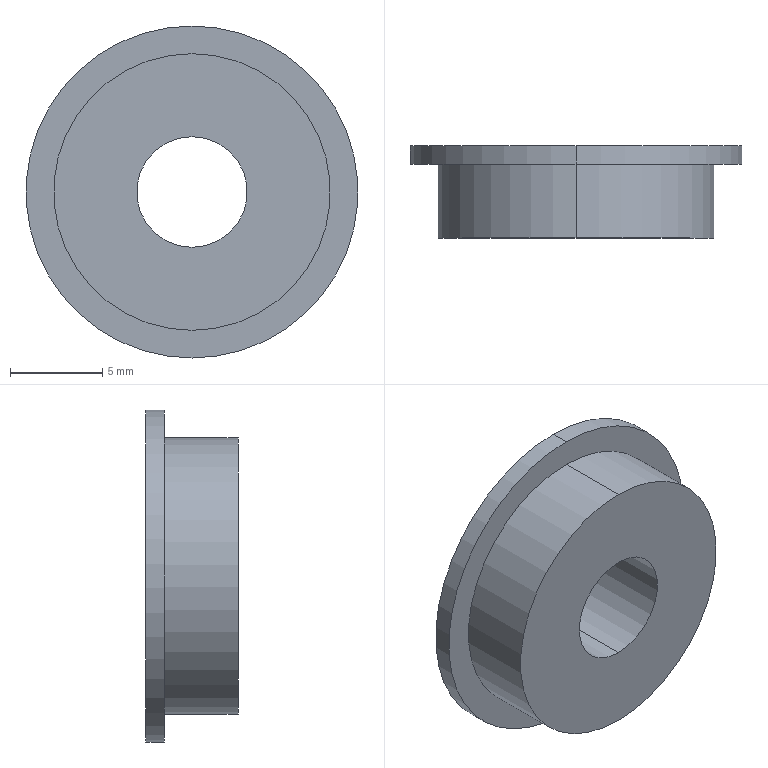Component | SolidWorks | 6 15 5 F-2 | 1 solid | 9 faces | box 18 x 5 x 18 mm | volume 820 mm3 | cylinder 6 | plane 3 | commonest cylinder face diameters 18 x2 6 x2 15 x2
build123d program:
from build123d import *

# Parameters (mm, degrees)
SKETCH1_R           = 7.5
SKETCH1_R_2         = 3
BOSS_EXTRUDE1_DEPTH = 5
BOSS_EXTRUDE2_START = -1
SKETCH2_R           = 9
SKETCH2_R_2         = 3
BOSS_EXTRUDE2_DEPTH = 1


with BuildPart() as part:
    # Sketch1 → Boss-Extrude1 (new body)
    with BuildSketch(Plane(origin=(0, 0, 0), x_dir=(1, 0, 0), z_dir=(0, 1, 0))):
        with Locations(Location((0, 0, 0), (0, 0, 270))):
            Circle(SKETCH1_R)
        with Locations(Location((0, 0, 0), (0, 0, 270))):
            Circle(SKETCH1_R_2, mode=Mode.SUBTRACT)
    extrude(amount=BOSS_EXTRUDE1_DEPTH)

    # Sketch2 → Boss-Extrude2 (add)
    with BuildSketch(Plane(origin=(0, 5, 0), x_dir=(1, 0, 0), z_dir=(0, 1, 0)).offset(BOSS_EXTRUDE2_START)):
        with Locations(Location((0, 0, 0), (0, 0, 270))):
            Circle(SKETCH2_R)
        with Locations(Location((0, 0, 0), (0, 0, 270))):
            Circle(SKETCH2_R_2, mode=Mode.SUBTRACT)
    extrude(amount=BOSS_EXTRUDE2_DEPTH)


solid = part.part

# Placed as in the assembly
solid = solid.moved(Location((0.3183, -14.6, 37), (0, 0, 0)))
STEP:
#1=COLOUR_RGB('',0.7922,0.8196,0.9333);
#2=FILL_AREA_STYLE_COLOUR('',#1);
#3=FILL_AREA_STYLE('',(#2));
#4=SURFACE_STYLE_FILL_AREA(#3);
#5=SURFACE_SIDE_STYLE('',(#4));
#6=SURFACE_STYLE_USAGE(.BOTH.,#5);
#7=PRESENTATION_STYLE_ASSIGNMENT((#6));
#8=CARTESIAN_POINT('',(0.01253,-0.4173,1.811));
#9=VERTEX_POINT('',#8);
#10=CARTESIAN_POINT('',(0.01253,-0.4173,1.102));
#11=VERTEX_POINT('',#10);
#12=CARTESIAN_POINT('',(0.01253,-0.4173,1.457));
#13=DIRECTION('',(0.,1.,0.));
#14=DIRECTION('',(0.,0.,1.));
#15=AXIS2_PLACEMENT_3D('',#12,#13,#14);
#16=CIRCLE('',#15,0.3543);
#17=EDGE_CURVE('',#9,#11,#16,.T.);
#18=ORIENTED_EDGE('',*,*,#17,.T.);
#19=CARTESIAN_POINT('',(0.01253,-0.378,1.102));
#20=VERTEX_POINT('',#19);
#21=CARTESIAN_POINT('',(0.01253,-0.4173,1.102));
#22=DIRECTION('',(0.,1.,0.));
#23=VECTOR('',#22,39.37);
#24=LINE('',#21,#23);
#25=EDGE_CURVE('',#11,#20,#24,.T.);
#26=ORIENTED_EDGE('',*,*,#25,.T.);
#27=CARTESIAN_POINT('',(0.01253,-0.378,1.811));
#28=VERTEX_POINT('',#27);
#29=CARTESIAN_POINT('',(0.01253,-0.378,1.457));
#30=DIRECTION('',(0.,1.,0.));
#31=DIRECTION('',(0.,0.,1.));
#32=AXIS2_PLACEMENT_3D('',#29,#30,#31);
#33=CIRCLE('',#32,0.3543);
#34=EDGE_CURVE('',#28,#20,#33,.T.);
#35=ORIENTED_EDGE('',*,*,#34,.F.);
#36=CARTESIAN_POINT('',(0.01253,-0.4173,1.811));
#37=DIRECTION('',(0.,1.,0.));
#38=VECTOR('',#37,39.37);
#39=LINE('',#36,#38);
#40=EDGE_CURVE('',#9,#28,#39,.T.);
#41=ORIENTED_EDGE('',*,*,#40,.F.);
#42=EDGE_LOOP('',(#18,#26,#35,#41));
#43=FACE_OUTER_BOUND('',#42,.T.);
#44=CARTESIAN_POINT('',(0.01253,-0.4173,1.457));
#45=DIRECTION('',(0.,1.,0.));
#46=DIRECTION('',(0.,0.,1.));
#47=AXIS2_PLACEMENT_3D('',#44,#45,#46);
#48=CYLINDRICAL_SURFACE('',#47,0.3543);
#49=ADVANCED_FACE('',(#43),#48,.T.);
#50=CARTESIAN_POINT('',(0.01253,-0.378,1.339));
#51=VERTEX_POINT('',#50);
#52=CARTESIAN_POINT('',(0.01253,-0.378,1.575));
#53=VERTEX_POINT('',#52);
#54=CARTESIAN_POINT('',(0.01253,-0.378,1.457));
#55=DIRECTION('',(0.,1.,0.));
#56=DIRECTION('',(0.,0.,1.));
#57=AXIS2_PLACEMENT_3D('',#54,#55,#56);
#58=CIRCLE('',#57,0.1181);
#59=EDGE_CURVE('',#51,#53,#58,.T.);
#60=ORIENTED_EDGE('',*,*,#59,.T.);
#61=CARTESIAN_POINT('',(0.01253,-0.5748,1.575));
#62=VERTEX_POINT('',#61);
#63=CARTESIAN_POINT('',(0.01253,-0.378,1.575));
#64=DIRECTION('',(0.,-1.,0.));
#65=VECTOR('',#64,39.37);
#66=LINE('',#63,#65);
#67=EDGE_CURVE('',#53,#62,#66,.T.);
#68=ORIENTED_EDGE('',*,*,#67,.T.);
#69=CARTESIAN_POINT('',(0.01253,-0.5748,1.339));
#70=VERTEX_POINT('',#69);
#71=CARTESIAN_POINT('',(0.01253,-0.5748,1.457));
#72=DIRECTION('',(0.,1.,0.));
#73=DIRECTION('',(0.,0.,1.));
#74=AXIS2_PLACEMENT_3D('',#71,#72,#73);
#75=CIRCLE('',#74,0.1181);
#76=EDGE_CURVE('',#70,#62,#75,.T.);
#77=ORIENTED_EDGE('',*,*,#76,.F.);
#78=CARTESIAN_POINT('',(0.01253,-0.378,1.339));
#79=DIRECTION('',(0.,-1.,0.));
#80=VECTOR('',#79,39.37);
#81=LINE('',#78,#80);
#82=EDGE_CURVE('',#51,#70,#81,.T.);
#83=ORIENTED_EDGE('',*,*,#82,.F.);
#84=EDGE_LOOP('',(#60,#68,#77,#83));
#85=FACE_OUTER_BOUND('',#84,.T.);
#86=CARTESIAN_POINT('',(0.01253,-0.378,1.457));
#87=DIRECTION('',(0.,-1.,0.));
#88=DIRECTION('',(0.,0.,-1.));
#89=AXIS2_PLACEMENT_3D('',#86,#87,#88);
#90=CYLINDRICAL_SURFACE('',#89,0.1181);
#91=ADVANCED_FACE('',(#85),#90,.F.);
#92=CARTESIAN_POINT('',(0.01253,-0.4173,1.752));
#93=VERTEX_POINT('',#92);
#94=CARTESIAN_POINT('',(0.01253,-0.4173,1.161));
#95=VERTEX_POINT('',#94);
#96=CARTESIAN_POINT('',(0.01253,-0.4173,1.457));
#97=DIRECTION('',(0.,1.,0.));
#98=DIRECTION('',(0.,0.,1.));
#99=AXIS2_PLACEMENT_3D('',#96,#97,#98);
#100=CIRCLE('',#99,0.2953);
#101=EDGE_CURVE('',#93,#95,#100,.T.);
#102=ORIENTED_EDGE('',*,*,#101,.F.);
#103=CARTESIAN_POINT('',(0.01253,-0.5748,1.752));
#104=VERTEX_POINT('',#103);
#105=CARTESIAN_POINT('',(0.01253,-0.378,1.752));
#106=DIRECTION('',(0.,-1.,0.));
#107=VECTOR('',#106,39.37);
#108=LINE('',#105,#107);
#109=EDGE_CURVE('',#93,#104,#108,.T.);
#110=ORIENTED_EDGE('',*,*,#109,.T.);
#111=CARTESIAN_POINT('',(0.01253,-0.5748,1.161));
#112=VERTEX_POINT('',#111);
#113=CARTESIAN_POINT('',(0.01253,-0.5748,1.457));
#114=DIRECTION('',(0.,1.,0.));
#115=DIRECTION('',(0.,0.,1.));
#116=AXIS2_PLACEMENT_3D('',#113,#114,#115);
#117=CIRCLE('',#116,0.2953);
#118=EDGE_CURVE('',#104,#112,#117,.T.);
#119=ORIENTED_EDGE('',*,*,#118,.T.);
#120=CARTESIAN_POINT('',(0.01253,-0.378,1.161));
#121=DIRECTION('',(0.,-1.,0.));
#122=VECTOR('',#121,39.37);
#123=LINE('',#120,#122);
#124=EDGE_CURVE('',#95,#112,#123,.T.);
#125=ORIENTED_EDGE('',*,*,#124,.F.);
#126=EDGE_LOOP('',(#102,#110,#119,#125));
#127=FACE_OUTER_BOUND('',#126,.T.);
#128=CARTESIAN_POINT('',(0.01253,-0.378,1.457));
#129=DIRECTION('',(0.,-1.,0.));
#130=DIRECTION('',(0.,0.,-1.));
#131=AXIS2_PLACEMENT_3D('',#128,#129,#130);
#132=CYLINDRICAL_SURFACE('',#131,0.2953);
#133=ADVANCED_FACE('',(#127),#132,.T.);
#134=ORIENTED_EDGE('',*,*,#109,.F.);
#135=CARTESIAN_POINT('',(0.01253,-0.4173,1.457));
#136=DIRECTION('',(0.,1.,0.));
#137=DIRECTION('',(0.,0.,1.));
#138=AXIS2_PLACEMENT_3D('',#135,#136,#137);
#139=CIRCLE('',#138,0.2953);
#140=EDGE_CURVE('',#95,#93,#139,.T.);
#141=ORIENTED_EDGE('',*,*,#140,.F.);
#142=ORIENTED_EDGE('',*,*,#124,.T.);
#143=CARTESIAN_POINT('',(0.01253,-0.5748,1.457));
#144=DIRECTION('',(0.,1.,0.));
#145=DIRECTION('',(0.,0.,1.));
#146=AXIS2_PLACEMENT_3D('',#143,#144,#145);
#147=CIRCLE('',#146,0.2953);
#148=EDGE_CURVE('',#112,#104,#147,.T.);
#149=ORIENTED_EDGE('',*,*,#148,.T.);
#150=EDGE_LOOP('',(#134,#141,#142,#149));
#151=FACE_OUTER_BOUND('',#150,.T.);
#152=CARTESIAN_POINT('',(0.01253,-0.378,1.457));
#153=DIRECTION('',(0.,-1.,0.));
#154=DIRECTION('',(0.,0.,-1.));
#155=AXIS2_PLACEMENT_3D('',#152,#153,#154);
#156=CYLINDRICAL_SURFACE('',#155,0.2953);
#157=ADVANCED_FACE('',(#151),#156,.T.);
#158=ORIENTED_EDGE('',*,*,#59,.F.);
#159=CARTESIAN_POINT('',(0.01253,-0.378,1.457));
#160=DIRECTION('',(0.,1.,0.));
#161=DIRECTION('',(0.,0.,1.));
#162=AXIS2_PLACEMENT_3D('',#159,#160,#161);
#163=CIRCLE('',#162,0.1181);
#164=EDGE_CURVE('',#53,#51,#163,.T.);
#165=ORIENTED_EDGE('',*,*,#164,.F.);
#166=EDGE_LOOP('',(#158,#165));
#167=FACE_BOUND('',#166,.T.);
#168=ORIENTED_EDGE('',*,*,#34,.T.);
#169=CARTESIAN_POINT('',(0.01253,-0.378,1.457));
#170=DIRECTION('',(0.,1.,0.));
#171=DIRECTION('',(0.,0.,1.));
#172=AXIS2_PLACEMENT_3D('',#169,#170,#171);
#173=CIRCLE('',#172,0.3543);
#174=EDGE_CURVE('',#20,#28,#173,.T.);
#175=ORIENTED_EDGE('',*,*,#174,.T.);
#176=EDGE_LOOP('',(#168,#175));
#177=FACE_OUTER_BOUND('',#176,.T.);
#178=CARTESIAN_POINT('',(0.01253,-0.378,1.457));
#179=DIRECTION('',(0.,1.,0.));
#180=DIRECTION('',(0.,0.,1.));
#181=AXIS2_PLACEMENT_3D('',#178,#179,#180);
#182=PLANE('',#181);
#183=ADVANCED_FACE('',(#167,#177),#182,.T.);
#184=ORIENTED_EDGE('',*,*,#148,.F.);
#185=ORIENTED_EDGE('',*,*,#118,.F.);
#186=EDGE_LOOP('',(#184,#185));
#187=FACE_OUTER_BOUND('',#186,.T.);
#188=ORIENTED_EDGE('',*,*,#76,.T.);
#189=CARTESIAN_POINT('',(0.01253,-0.5748,1.457));
#190=DIRECTION('',(0.,1.,0.));
#191=DIRECTION('',(0.,0.,1.));
#192=AXIS2_PLACEMENT_3D('',#189,#190,#191);
#193=CIRCLE('',#192,0.1181);
#194=EDGE_CURVE('',#62,#70,#193,.T.);
#195=ORIENTED_EDGE('',*,*,#194,.T.);
#196=EDGE_LOOP('',(#188,#195));
#197=FACE_BOUND('',#196,.T.);
#198=CARTESIAN_POINT('',(0.01253,-0.5748,1.457));
#199=DIRECTION('',(0.,1.,0.));
#200=DIRECTION('',(0.,0.,1.));
#201=AXIS2_PLACEMENT_3D('',#198,#199,#200);
#202=PLANE('',#201);
#203=ADVANCED_FACE('',(#187,#197),#202,.F.);
#204=ORIENTED_EDGE('',*,*,#67,.F.);
#205=ORIENTED_EDGE('',*,*,#164,.T.);
#206=ORIENTED_EDGE('',*,*,#82,.T.);
#207=ORIENTED_EDGE('',*,*,#194,.F.);
#208=EDGE_LOOP('',(#204,#205,#206,#207));
#209=FACE_OUTER_BOUND('',#208,.T.);
#210=CARTESIAN_POINT('',(0.01253,-0.378,1.457));
#211=DIRECTION('',(0.,-1.,0.));
#212=DIRECTION('',(0.,0.,-1.));
#213=AXIS2_PLACEMENT_3D('',#210,#211,#212);
#214=CYLINDRICAL_SURFACE('',#213,0.1181);
#215=ADVANCED_FACE('',(#209),#214,.F.);
#216=ORIENTED_EDGE('',*,*,#17,.F.);
#217=CARTESIAN_POINT('',(0.01253,-0.4173,1.457));
#218=DIRECTION('',(0.,1.,0.));
#219=DIRECTION('',(0.,0.,1.));
#220=AXIS2_PLACEMENT_3D('',#217,#218,#219);
#221=CIRCLE('',#220,0.3543);
#222=EDGE_CURVE('',#11,#9,#221,.T.);
#223=ORIENTED_EDGE('',*,*,#222,.F.);
#224=EDGE_LOOP('',(#216,#223));
#225=FACE_OUTER_BOUND('',#224,.T.);
#226=ORIENTED_EDGE('',*,*,#140,.T.);
#227=ORIENTED_EDGE('',*,*,#101,.T.);
#228=EDGE_LOOP('',(#226,#227));
#229=FACE_BOUND('',#228,.T.);
#230=CARTESIAN_POINT('',(0.01253,-0.4173,1.457));
#231=DIRECTION('',(0.,1.,0.));
#232=DIRECTION('',(0.,0.,1.));
#233=AXIS2_PLACEMENT_3D('',#230,#231,#232);
#234=PLANE('',#233);
#235=ADVANCED_FACE('',(#225,#229),#234,.F.);
#236=ORIENTED_EDGE('',*,*,#25,.F.);
#237=ORIENTED_EDGE('',*,*,#222,.T.);
#238=ORIENTED_EDGE('',*,*,#40,.T.);
#239=ORIENTED_EDGE('',*,*,#174,.F.);
#240=EDGE_LOOP('',(#236,#237,#238,#239));
#241=FACE_OUTER_BOUND('',#240,.T.);
#242=CARTESIAN_POINT('',(0.01253,-0.4173,1.457));
#243=DIRECTION('',(0.,1.,0.));
#244=DIRECTION('',(0.,0.,1.));
#245=AXIS2_PLACEMENT_3D('',#242,#243,#244);
#246=CYLINDRICAL_SURFACE('',#245,0.3543);
#247=ADVANCED_FACE('',(#241),#246,.T.);
#248=CLOSED_SHELL('',(#49,#91,#133,#157,#183,#203,#215,#235,#247));
#249=MANIFOLD_SOLID_BREP('',#248);
#250=STYLED_ITEM('',(#7),#249);
#251=PRESENTATION_LAYER_ASSIGNMENT('','',(#250));
#252=(LENGTH_UNIT()NAMED_UNIT(*)SI_UNIT($,.METRE.));
#253=LENGTH_MEASURE_WITH_UNIT(LENGTH_MEASURE(0.0254),#252);
#254=DIMENSIONAL_EXPONENTS(1.,0.,0.,0.,0.,0.,0.);
#255=(CONVERSION_BASED_UNIT('',#253)LENGTH_UNIT()NAMED_UNIT(#254));
#256=UNCERTAINTY_MEASURE_WITH_UNIT(LENGTH_MEASURE(0.00001),#255,'','');
#257=(NAMED_UNIT(*)PLANE_ANGLE_UNIT()SI_UNIT($,.RADIAN.));
#258=(NAMED_UNIT(*)SI_UNIT($,.STERADIAN.)SOLID_ANGLE_UNIT());
#259=(GEOMETRIC_REPRESENTATION_CONTEXT(3)GLOBAL_UNCERTAINTY_ASSIGNED_CONTEXT((#256))GLOBAL_UNIT_ASSIGNED_CONTEXT((#255,#257,#258))REPRESENTATION_CONTEXT('',''));
#260=MECHANICAL_DESIGN_GEOMETRIC_PRESENTATION_REPRESENTATION('',(#250),#259);
#261=CARTESIAN_POINT('',(0.,0.,0.));
#262=DIRECTION('',(0.,0.,1.));
#263=DIRECTION('',(1.,0.,0.));
#264=AXIS2_PLACEMENT_3D('',#261,#262,#263);
#265=(LENGTH_UNIT()NAMED_UNIT(*)SI_UNIT($,.METRE.));
#266=LENGTH_MEASURE_WITH_UNIT(LENGTH_MEASURE(0.0254),#265);
#267=DIMENSIONAL_EXPONENTS(1.,0.,0.,0.,0.,0.,0.);
#268=(CONVERSION_BASED_UNIT('',#266)LENGTH_UNIT()NAMED_UNIT(#267));
#269=UNCERTAINTY_MEASURE_WITH_UNIT(LENGTH_MEASURE(0.00001),#268,'','');
#270=(NAMED_UNIT(*)PLANE_ANGLE_UNIT()SI_UNIT($,.RADIAN.));
#271=(NAMED_UNIT(*)SI_UNIT($,.STERADIAN.)SOLID_ANGLE_UNIT());
#272=(GEOMETRIC_REPRESENTATION_CONTEXT(3)GLOBAL_UNCERTAINTY_ASSIGNED_CONTEXT((#269))GLOBAL_UNIT_ASSIGNED_CONTEXT((#268,#270,#271))REPRESENTATION_CONTEXT('',''));
#273=ADVANCED_BREP_SHAPE_REPRESENTATION('',(#249,#264),#272);